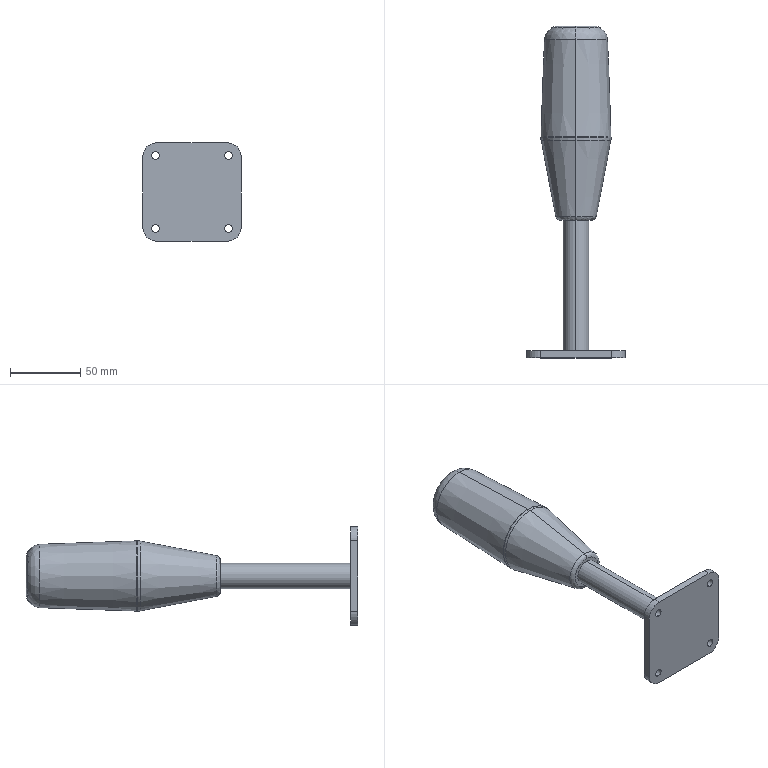Component | SolidWorks | 50MMRodThree-ColorLight-1 | 1 solid | 38 faces | volume 255843 mm3 | cylinder 14 | spline 10 | plane 8 | cone 6 | commonest cylinder face diameters 5.5 x8 20 x4 18 x2